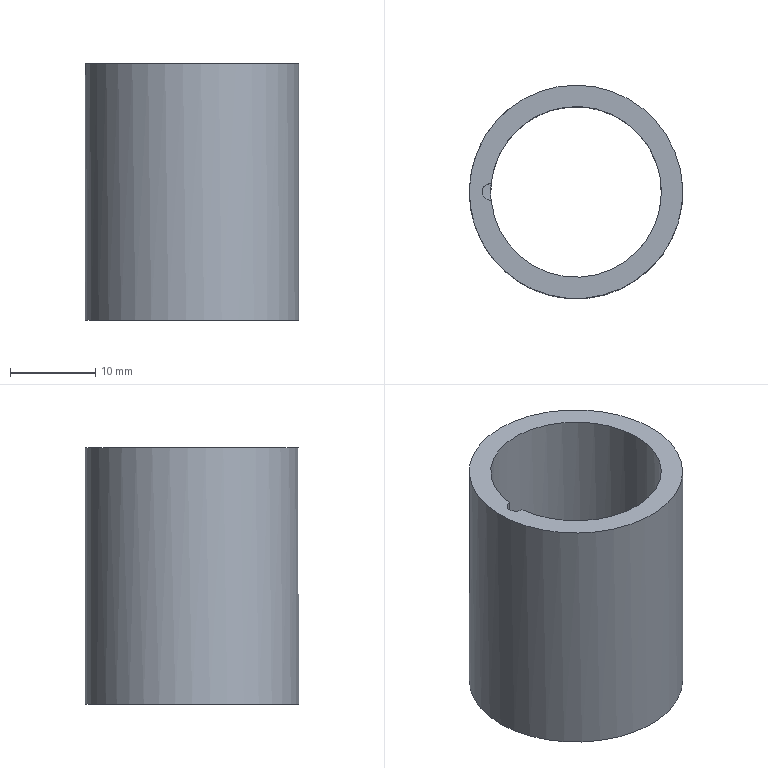Component | NX | 7_BUSHING | 1 solid | 6 faces | volume 5138 mm3 | cylinder 3 | cone 2 | plane 1 | commonest cylinder face diameters 25 x1 20 x1 2 x1